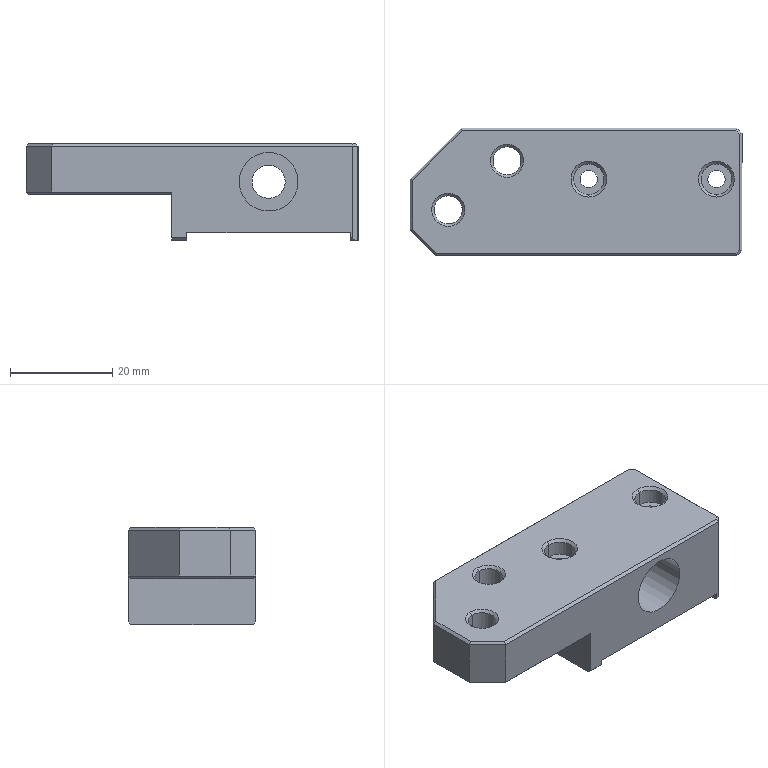Component | SolidWorks | UpperRollerFixedSeat-1 | 1 solid | 66 faces | volume 19493 mm3 | plane 38 | cylinder 20 | cone 8 | commonest cylinder face diameters 5.5 x4 6 x4 10 x4 3.4 x4 11.5 x2 6.5 x2